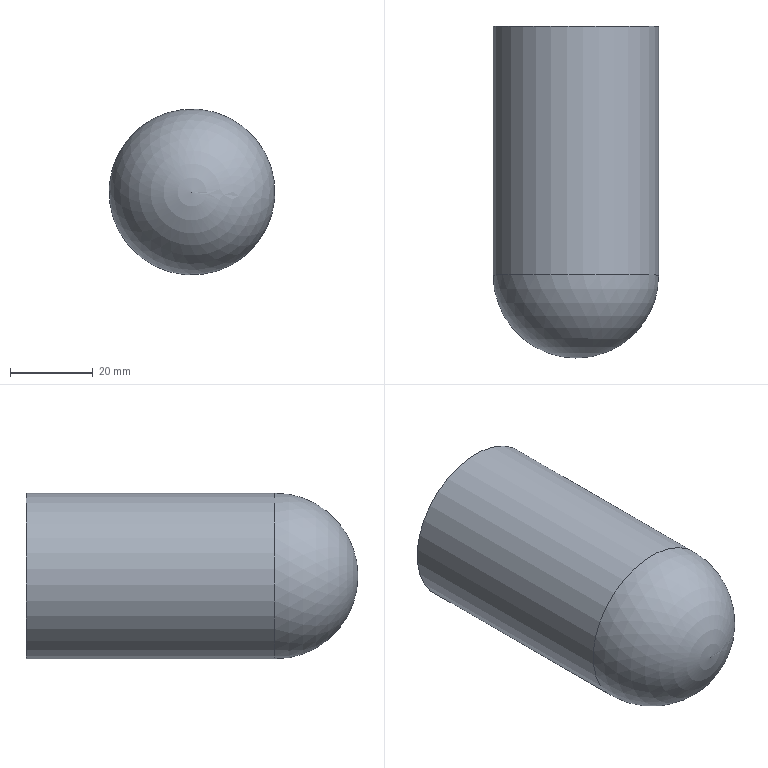Component | NX | TOP_SHELL | 1 solid | 5 faces | box 40 x 80 x 40 mm | volume 65544 mm3 | cylinder 2 | plane 2 | sphere 1 | commonest cylinder face diameters 22 x1 40 x1
STEP:
#1=CARTESIAN_POINT('',(0.,0.,0.));
#2=DIRECTION('',(0.,0.,1.));
#3=DIRECTION('',(1.,0.,0.));
#4=AXIS2_PLACEMENT_3D('',#1,#2,#3);
#5=CARTESIAN_POINT('',(-20.87,-81.911,-10.958));
#6=VERTEX_POINT('',#5);
#7=CARTESIAN_POINT('',(-19.911,-81.911,-0.));
#8=DIRECTION('',(0.,1.,0.));
#9=DIRECTION('',(-0.08716,0.,-0.9962));
#10=AXIS2_PLACEMENT_3D('',#7,#8,#9);
#11=CIRCLE('',#10,11.);
#12=CARTESIAN_POINT('',(-19.911,-81.911,-0.));
#13=DIRECTION('',(0.,-1.,0.));
#14=DIRECTION('',(-0.9962,0.,0.08716));
#15=AXIS2_PLACEMENT_3D('',#12,#13,#14);
#16=CYLINDRICAL_SURFACE('',#15,11.);
#17=CARTESIAN_POINT('',(7.854,0.));
#18=DIRECTION('',(-1.,0.));
#19=VECTOR('',#18,1.);
#20=LINE('',#17,#19);
#21=(GEOMETRIC_REPRESENTATION_CONTEXT(2)PARAMETRIC_REPRESENTATION_CONTEXT()REPRESENTATION_CONTEXT('',''));
#22=DEFINITIONAL_REPRESENTATION('',(#20),#21);
#23=PCURVE('',#16,#22);
#24=CARTESIAN_POINT('',(-19.911,-81.911,-0.));
#25=DIRECTION('',(0.,1.,0.));
#26=DIRECTION('',(0.9962,0.,-0.08716));
#27=AXIS2_PLACEMENT_3D('',#24,#25,#26);
#28=PLANE('',#27);
#29=CARTESIAN_POINT('',(0.,0.));
#30=DIRECTION('',(0.,1.));
#31=AXIS2_PLACEMENT_2D('',#29,#30);
#32=CIRCLE('',#31,11.);
#33=(GEOMETRIC_REPRESENTATION_CONTEXT(2)PARAMETRIC_REPRESENTATION_CONTEXT()REPRESENTATION_CONTEXT('',''));
#34=DEFINITIONAL_REPRESENTATION('',(#32),#33);
#35=PCURVE('',#28,#34);
#36=SURFACE_CURVE('',#11,(#23,#35),.PCURVE_S1.);
#37=EDGE_CURVE('',#6,#6,#36,.T.);
#38=ORIENTED_EDGE('',*,*,#37,.F.);
#39=CARTESIAN_POINT('',(-20.87,-151.911,-10.958));
#40=VERTEX_POINT('',#39);
#41=CARTESIAN_POINT('',(-20.87,-81.911,-10.958));
#42=CARTESIAN_POINT('',(-20.87,-151.911,-10.958));
#43=B_SPLINE_CURVE_WITH_KNOTS('',1,(#41,#42),.UNSPECIFIED.,.F.,.F.,(2,2),(0.,70.),.PIECEWISE_BEZIER_KNOTS.);
#44=CARTESIAN_POINT('',(7.854,0.));
#45=DIRECTION('',(0.,1.));
#46=VECTOR('',#45,1.);
#47=LINE('',#44,#46);
#48=(GEOMETRIC_REPRESENTATION_CONTEXT(2)PARAMETRIC_REPRESENTATION_CONTEXT()REPRESENTATION_CONTEXT('',''));
#49=DEFINITIONAL_REPRESENTATION('',(#47),#48);
#50=PCURVE('',#16,#49);
#51=CARTESIAN_POINT('',(1.571,0.));
#52=DIRECTION('',(0.,1.));
#53=VECTOR('',#52,1.);
#54=LINE('',#51,#53);
#55=(GEOMETRIC_REPRESENTATION_CONTEXT(2)PARAMETRIC_REPRESENTATION_CONTEXT()REPRESENTATION_CONTEXT('',''));
#56=DEFINITIONAL_REPRESENTATION('',(#54),#55);
#57=PCURVE('',#16,#56);
#58=SEAM_CURVE('',#43,(#50,#57),.PCURVE_S1.);
#59=EDGE_CURVE('',#6,#40,#58,.T.);
#60=ORIENTED_EDGE('',*,*,#59,.T.);
#61=CARTESIAN_POINT('',(-19.911,-151.911,-0.));
#62=DIRECTION('',(0.,-1.,0.));
#63=DIRECTION('',(-0.08716,0.,-0.9962));
#64=AXIS2_PLACEMENT_3D('',#61,#62,#63);
#65=CIRCLE('',#64,11.);
#66=CARTESIAN_POINT('',(1.571,70.));
#67=DIRECTION('',(1.,0.));
#68=VECTOR('',#67,1.);
#69=LINE('',#66,#68);
#70=(GEOMETRIC_REPRESENTATION_CONTEXT(2)PARAMETRIC_REPRESENTATION_CONTEXT()REPRESENTATION_CONTEXT('',''));
#71=DEFINITIONAL_REPRESENTATION('',(#69),#70);
#72=PCURVE('',#16,#71);
#73=CARTESIAN_POINT('',(-19.911,-151.911,-0.));
#74=DIRECTION('',(0.,-1.,0.));
#75=DIRECTION('',(-0.9962,0.,0.08716));
#76=AXIS2_PLACEMENT_3D('',#73,#74,#75);
#77=PLANE('',#76);
#78=CARTESIAN_POINT('',(0.,0.));
#79=DIRECTION('',(0.,1.));
#80=AXIS2_PLACEMENT_2D('',#78,#79);
#81=CIRCLE('',#80,11.);
#82=(GEOMETRIC_REPRESENTATION_CONTEXT(2)PARAMETRIC_REPRESENTATION_CONTEXT()REPRESENTATION_CONTEXT('',''));
#83=DEFINITIONAL_REPRESENTATION('',(#81),#82);
#84=PCURVE('',#77,#83);
#85=SURFACE_CURVE('',#65,(#72,#84),.PCURVE_S1.);
#86=EDGE_CURVE('',#40,#40,#85,.T.);
#87=ORIENTED_EDGE('',*,*,#86,.F.);
#88=ORIENTED_EDGE('',*,*,#59,.F.);
#89=EDGE_LOOP('',(#38,#60,#87,#88));
#90=FACE_BOUND('',#89,.F.);
#91=ADVANCED_FACE('',(#90),#16,.F.);
#92=CARTESIAN_POINT('',(-39.835,-141.911,1.743));
#93=VERTEX_POINT('',#92);
#94=CARTESIAN_POINT('',(0.01289,-141.911,-1.743));
#95=VERTEX_POINT('',#94);
#96=CARTESIAN_POINT('',(-19.911,-141.911,-0.));
#97=DIRECTION('',(0.,1.,0.));
#98=DIRECTION('',(-0.9962,0.,0.08716));
#99=AXIS2_PLACEMENT_3D('',#96,#97,#98);
#100=CIRCLE('',#99,20.);
#101=CARTESIAN_POINT('',(-19.911,-81.911,-0.));
#102=DIRECTION('',(0.,-1.,0.));
#103=DIRECTION('',(-0.9962,0.,0.08716));
#104=AXIS2_PLACEMENT_3D('',#101,#102,#103);
#105=CYLINDRICAL_SURFACE('',#104,20.);
#106=CARTESIAN_POINT('',(6.283,60.));
#107=DIRECTION('',(-1.,0.));
#108=VECTOR('',#107,1.);
#109=LINE('',#106,#108);
#110=(GEOMETRIC_REPRESENTATION_CONTEXT(2)PARAMETRIC_REPRESENTATION_CONTEXT()REPRESENTATION_CONTEXT('',''));
#111=DEFINITIONAL_REPRESENTATION('',(#109),#110);
#112=PCURVE('',#105,#111);
#113=CARTESIAN_POINT('',(-19.911,-141.911,-0.));
#114=DIRECTION('',(0.,1.,-0.));
#115=DIRECTION('',(0.9962,-0.,-0.08716));
#116=AXIS2_PLACEMENT_3D('',#113,#114,#115);
#117=SPHERICAL_SURFACE('',#116,20.);
#118=CARTESIAN_POINT('',(3.142,0.));
#119=CARTESIAN_POINT('',(3.237,0.));
#120=CARTESIAN_POINT('',(3.427,0.));
#121=CARTESIAN_POINT('',(3.713,0.));
#122=CARTESIAN_POINT('',(3.998,0.));
#123=CARTESIAN_POINT('',(4.284,0.));
#124=CARTESIAN_POINT('',(4.57,0.));
#125=CARTESIAN_POINT('',(4.855,0.));
#126=CARTESIAN_POINT('',(5.141,0.));
#127=CARTESIAN_POINT('',(5.426,0.));
#128=CARTESIAN_POINT('',(5.712,0.));
#129=CARTESIAN_POINT('',(5.998,0.));
#130=CARTESIAN_POINT('',(6.283,0.));
#131=CARTESIAN_POINT('',(6.569,0.));
#132=CARTESIAN_POINT('',(6.854,0.));
#133=CARTESIAN_POINT('',(7.14,0.));
#134=CARTESIAN_POINT('',(7.426,0.));
#135=CARTESIAN_POINT('',(7.711,0.));
#136=CARTESIAN_POINT('',(7.997,0.));
#137=CARTESIAN_POINT('',(8.282,0.));
#138=CARTESIAN_POINT('',(8.568,0.));
#139=CARTESIAN_POINT('',(8.854,0.));
#140=CARTESIAN_POINT('',(9.139,0.));
#141=CARTESIAN_POINT('',(9.33,0.));
#142=CARTESIAN_POINT('',(9.425,0.));
#143=B_SPLINE_CURVE_WITH_KNOTS('',3,(#118,#119,#120,#121,#122,#123,#124,#125,#126,#127,#128,#129,#130,#131,#132,#133,#134,#135,#136,#137,#138,#139,#140,#141,#142),.UNSPECIFIED.,.F.,.F.,(4,1,1,1,1,1,1,1,1,1,1,1,1,1,1,1,1,1,1,1,1,1,4),(0.,0.2856,0.5712,0.8568,1.142,1.428,1.714,1.999,2.285,2.57,2.856,3.142,3.427,3.713,3.998,4.284,4.57,4.855,5.141,5.426,5.712,5.998,6.283),.QUASI_UNIFORM_KNOTS.);
#144=(GEOMETRIC_REPRESENTATION_CONTEXT(2)PARAMETRIC_REPRESENTATION_CONTEXT()REPRESENTATION_CONTEXT('',''));
#145=DEFINITIONAL_REPRESENTATION('',(#143),#144);
#146=PCURVE('',#117,#145);
#147=SURFACE_CURVE('',#100,(#112,#146),.PCURVE_S1.);
#148=EDGE_CURVE('',#93,#95,#147,.T.);
#149=ORIENTED_EDGE('',*,*,#148,.T.);
#150=CARTESIAN_POINT('',(-19.911,-141.911,-0.));
#151=DIRECTION('',(0.,1.,0.));
#152=DIRECTION('',(-0.9962,0.,0.08716));
#153=AXIS2_PLACEMENT_3D('',#150,#151,#152);
#154=CIRCLE('',#153,20.);
#155=CARTESIAN_POINT('',(6.283,60.));
#156=DIRECTION('',(-1.,0.));
#157=VECTOR('',#156,1.);
#158=LINE('',#155,#157);
#159=(GEOMETRIC_REPRESENTATION_CONTEXT(2)PARAMETRIC_REPRESENTATION_CONTEXT()REPRESENTATION_CONTEXT('',''));
#160=DEFINITIONAL_REPRESENTATION('',(#158),#159);
#161=PCURVE('',#105,#160);
#162=CARTESIAN_POINT('',(-3.142,0.));
#163=CARTESIAN_POINT('',(-3.046,0.));
#164=CARTESIAN_POINT('',(-2.856,0.));
#165=CARTESIAN_POINT('',(-2.57,0.));
#166=CARTESIAN_POINT('',(-2.285,0.));
#167=CARTESIAN_POINT('',(-1.999,0.));
#168=CARTESIAN_POINT('',(-1.714,0.));
#169=CARTESIAN_POINT('',(-1.428,0.));
#170=CARTESIAN_POINT('',(-1.142,0.));
#171=CARTESIAN_POINT('',(-0.8568,0.));
#172=CARTESIAN_POINT('',(-0.5712,0.));
#173=CARTESIAN_POINT('',(-0.2856,0.));
#174=CARTESIAN_POINT('',(0.,0.));
#175=CARTESIAN_POINT('',(0.2856,0.));
#176=CARTESIAN_POINT('',(0.5712,0.));
#177=CARTESIAN_POINT('',(0.8568,0.));
#178=CARTESIAN_POINT('',(1.142,0.));
#179=CARTESIAN_POINT('',(1.428,0.));
#180=CARTESIAN_POINT('',(1.714,0.));
#181=CARTESIAN_POINT('',(1.999,0.));
#182=CARTESIAN_POINT('',(2.285,0.));
#183=CARTESIAN_POINT('',(2.57,0.));
#184=CARTESIAN_POINT('',(2.856,0.));
#185=CARTESIAN_POINT('',(3.046,0.));
#186=CARTESIAN_POINT('',(3.142,0.));
#187=B_SPLINE_CURVE_WITH_KNOTS('',3,(#162,#163,#164,#165,#166,#167,#168,#169,#170,#171,#172,#173,#174,#175,#176,#177,#178,#179,#180,#181,#182,#183,#184,#185,#186),.UNSPECIFIED.,.F.,.F.,(4,1,1,1,1,1,1,1,1,1,1,1,1,1,1,1,1,1,1,1,1,1,4),(0.,0.2856,0.5712,0.8568,1.142,1.428,1.714,1.999,2.285,2.57,2.856,3.142,3.427,3.713,3.998,4.284,4.57,4.855,5.141,5.426,5.712,5.998,6.283),.QUASI_UNIFORM_KNOTS.);
#188=(GEOMETRIC_REPRESENTATION_CONTEXT(2)PARAMETRIC_REPRESENTATION_CONTEXT()REPRESENTATION_CONTEXT('',''));
#189=DEFINITIONAL_REPRESENTATION('',(#187),#188);
#190=PCURVE('',#117,#189);
#191=SURFACE_CURVE('',#154,(#161,#190),.PCURVE_S1.);
#192=EDGE_CURVE('',#95,#93,#191,.T.);
#193=ORIENTED_EDGE('',*,*,#192,.T.);
#194=CARTESIAN_POINT('',(-39.835,-81.911,1.743));
#195=VERTEX_POINT('',#194);
#196=CARTESIAN_POINT('',(-39.835,-81.911,1.743));
#197=CARTESIAN_POINT('',(-39.835,-141.911,1.743));
#198=B_SPLINE_CURVE_WITH_KNOTS('',1,(#196,#197),.UNSPECIFIED.,.F.,.F.,(2,2),(0.,60.),.PIECEWISE_BEZIER_KNOTS.);
#199=CARTESIAN_POINT('',(0.,0.));
#200=DIRECTION('',(0.,1.));
#201=VECTOR('',#200,1.);
#202=LINE('',#199,#201);
#203=(GEOMETRIC_REPRESENTATION_CONTEXT(2)PARAMETRIC_REPRESENTATION_CONTEXT()REPRESENTATION_CONTEXT('',''));
#204=DEFINITIONAL_REPRESENTATION('',(#202),#203);
#205=PCURVE('',#105,#204);
#206=CARTESIAN_POINT('',(6.283,0.));
#207=DIRECTION('',(0.,1.));
#208=VECTOR('',#207,1.);
#209=LINE('',#206,#208);
#210=(GEOMETRIC_REPRESENTATION_CONTEXT(2)PARAMETRIC_REPRESENTATION_CONTEXT()REPRESENTATION_CONTEXT('',''));
#211=DEFINITIONAL_REPRESENTATION('',(#209),#210);
#212=PCURVE('',#105,#211);
#213=SEAM_CURVE('',#198,(#205,#212),.PCURVE_S1.);
#214=EDGE_CURVE('',#195,#93,#213,.T.);
#215=ORIENTED_EDGE('',*,*,#214,.F.);
#216=CARTESIAN_POINT('',(-21.654,-81.911,-19.924));
#217=VERTEX_POINT('',#216);
#218=CARTESIAN_POINT('',(-19.911,-81.911,-0.));
#219=DIRECTION('',(0.,1.,0.));
#220=DIRECTION('',(-0.08716,0.,-0.9962));
#221=AXIS2_PLACEMENT_3D('',#218,#219,#220);
#222=CIRCLE('',#221,20.);
#223=CARTESIAN_POINT('',(1.571,0.));
#224=DIRECTION('',(-1.,0.));
#225=VECTOR('',#224,1.);
#226=LINE('',#223,#225);
#227=(GEOMETRIC_REPRESENTATION_CONTEXT(2)PARAMETRIC_REPRESENTATION_CONTEXT()REPRESENTATION_CONTEXT('',''));
#228=DEFINITIONAL_REPRESENTATION('',(#226),#227);
#229=PCURVE('',#105,#228);
#230=CARTESIAN_POINT('',(0.,0.));
#231=DIRECTION('',(0.,1.));
#232=AXIS2_PLACEMENT_2D('',#230,#231);
#233=CIRCLE('',#232,20.);
#234=(GEOMETRIC_REPRESENTATION_CONTEXT(2)PARAMETRIC_REPRESENTATION_CONTEXT()REPRESENTATION_CONTEXT('',''));
#235=DEFINITIONAL_REPRESENTATION('',(#233),#234);
#236=PCURVE('',#28,#235);
#237=SURFACE_CURVE('',#222,(#229,#236),.PCURVE_S1.);
#238=EDGE_CURVE('',#217,#195,#237,.T.);
#239=ORIENTED_EDGE('',*,*,#238,.F.);
#240=CARTESIAN_POINT('',(-19.911,-81.911,-0.));
#241=DIRECTION('',(0.,1.,0.));
#242=DIRECTION('',(-0.08716,0.,-0.9962));
#243=AXIS2_PLACEMENT_3D('',#240,#241,#242);
#244=CIRCLE('',#243,20.);
#245=CARTESIAN_POINT('',(7.854,0.));
#246=DIRECTION('',(-1.,0.));
#247=VECTOR('',#246,1.);
#248=LINE('',#245,#247);
#249=(GEOMETRIC_REPRESENTATION_CONTEXT(2)PARAMETRIC_REPRESENTATION_CONTEXT()REPRESENTATION_CONTEXT('',''));
#250=DEFINITIONAL_REPRESENTATION('',(#248),#249);
#251=PCURVE('',#105,#250);
#252=CARTESIAN_POINT('',(0.,0.));
#253=DIRECTION('',(0.,1.));
#254=AXIS2_PLACEMENT_2D('',#252,#253);
#255=CIRCLE('',#254,20.);
#256=(GEOMETRIC_REPRESENTATION_CONTEXT(2)PARAMETRIC_REPRESENTATION_CONTEXT()REPRESENTATION_CONTEXT('',''));
#257=DEFINITIONAL_REPRESENTATION('',(#255),#256);
#258=PCURVE('',#28,#257);
#259=SURFACE_CURVE('',#244,(#251,#258),.PCURVE_S1.);
#260=EDGE_CURVE('',#195,#217,#259,.T.);
#261=ORIENTED_EDGE('',*,*,#260,.F.);
#262=ORIENTED_EDGE('',*,*,#214,.T.);
#263=EDGE_LOOP('',(#149,#193,#215,#239,#261,#262));
#264=FACE_BOUND('',#263,.T.);
#265=ADVANCED_FACE('',(#264),#105,.T.);
#266=ORIENTED_EDGE('',*,*,#238,.T.);
#267=ORIENTED_EDGE('',*,*,#260,.T.);
#268=EDGE_LOOP('',(#266,#267));
#269=FACE_BOUND('',#268,.T.);
#270=ORIENTED_EDGE('',*,*,#37,.F.);
#271=EDGE_LOOP('',(#270));
#272=FACE_BOUND('',#271,.T.);
#273=ADVANCED_FACE('',(#269,#272),#28,.T.);
#274=ORIENTED_EDGE('',*,*,#86,.F.);
#275=EDGE_LOOP('',(#274));
#276=FACE_BOUND('',#275,.T.);
#277=ADVANCED_FACE('',(#276),#77,.F.);
#278=ORIENTED_EDGE('',*,*,#192,.F.);
#279=CARTESIAN_POINT('',(-19.911,-161.911,-0.));
#280=VERTEX_POINT('',#279);
#281=CARTESIAN_POINT('',(-19.911,-161.911,-0.));
#282=CARTESIAN_POINT('',(-15.44,-161.911,-0.3912));
#283=CARTESIAN_POINT('',(-10.969,-160.736,-0.7823));
#284=CARTESIAN_POINT('',(-6.866,-158.387,-1.141));
#285=CARTESIAN_POINT('',(-3.498,-155.006,-1.436));
#286=CARTESIAN_POINT('',(-1.158,-150.887,-1.641));
#287=CARTESIAN_POINT('',(0.01289,-146.399,-1.743));
#288=CARTESIAN_POINT('',(0.01289,-141.911,-1.743));
#289=B_SPLINE_CURVE_WITH_KNOTS('',7,(#281,#282,#283,#284,#285,#286,#287,#288),.UNSPECIFIED.,.F.,.F.,(8,8),(-1.571,0.),.PIECEWISE_BEZIER_KNOTS.);
#290=CARTESIAN_POINT('',(0.,0.));
#291=DIRECTION('',(0.,1.));
#292=VECTOR('',#291,1.);
#293=LINE('',#290,#292);
#294=(GEOMETRIC_REPRESENTATION_CONTEXT(2)PARAMETRIC_REPRESENTATION_CONTEXT()REPRESENTATION_CONTEXT('',''));
#295=DEFINITIONAL_REPRESENTATION('',(#293),#294);
#296=PCURVE('',#117,#295);
#297=CARTESIAN_POINT('',(6.283,0.));
#298=DIRECTION('',(0.,1.));
#299=VECTOR('',#298,1.);
#300=LINE('',#297,#299);
#301=(GEOMETRIC_REPRESENTATION_CONTEXT(2)PARAMETRIC_REPRESENTATION_CONTEXT()REPRESENTATION_CONTEXT('',''));
#302=DEFINITIONAL_REPRESENTATION('',(#300),#301);
#303=PCURVE('',#117,#302);
#304=SEAM_CURVE('',#289,(#296,#303),.PCURVE_S1.);
#305=EDGE_CURVE('',#280,#95,#304,.T.);
#306=ORIENTED_EDGE('',*,*,#305,.F.);
#307=ORIENTED_EDGE('',*,*,#305,.T.);
#308=ORIENTED_EDGE('',*,*,#148,.F.);
#309=EDGE_LOOP('',(#278,#306,#307,#308));
#310=FACE_BOUND('',#309,.T.);
#311=ADVANCED_FACE('',(#310),#117,.T.);
#312=CLOSED_SHELL('',(#91,#265,#273,#277,#311));
#313=MANIFOLD_SOLID_BREP('',#312);
#314=(LENGTH_UNIT()NAMED_UNIT(*)SI_UNIT(.MILLI.,.METRE.));
#315=UNCERTAINTY_MEASURE_WITH_UNIT(LENGTH_MEASURE(0.000005),#314,'','');
#316=(NAMED_UNIT(*)PLANE_ANGLE_UNIT()SI_UNIT($,.RADIAN.));
#317=(NAMED_UNIT(*)SI_UNIT($,.STERADIAN.)SOLID_ANGLE_UNIT());
#318=(GEOMETRIC_REPRESENTATION_CONTEXT(3)GLOBAL_UNCERTAINTY_ASSIGNED_CONTEXT((#315))GLOBAL_UNIT_ASSIGNED_CONTEXT((#314,#316,#317))REPRESENTATION_CONTEXT('',''));
#319=ADVANCED_BREP_SHAPE_REPRESENTATION('',(#4,#313),#318);